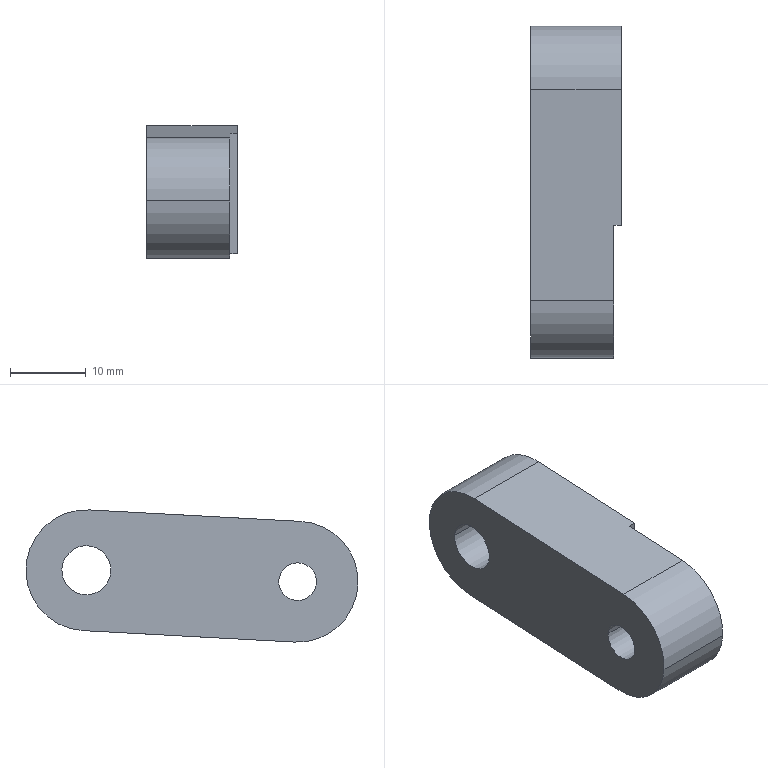Component | SolidWorks | NewDieSet-1_AdditionalStop-2 | 1 solid | 13 faces | box 12 x 43.96 x 17.51 mm | volume 6914 mm3 | cylinder 7 | plane 6 | commonest cylinder face diameters 16 x3 5 x2 6.5 x2
build123d program:
from build123d import *

# Parameters (mm, degrees)
BOSS_EXTRUDE1_DEPTH = 12
SKETCH2_R           = 3.25
CUT_EXTRUDE1_DEPTH  = 12
M6_TAPPED_HOLE1_D   = 5
SKETCH6_W           = 18
SKETCH6_H           = 1
CUT_EXTRUDE2_DEPTH  = 30.732


with BuildPart() as part:
    # Sketch1 → Boss-Extrude1 (new body)
    with BuildSketch(Plane(origin=(0, 0, 0), x_dir=(1, 0, 0), z_dir=(0, 1, 0))):
        with BuildLine():
            Line((-8, -14), (-8, 14))
            ThreePointArc((-8, 14), (0, 22), (8, 14))
            Line((8, 14), (8, -14))
            ThreePointArc((8, -14), (0, -22), (-8, -14))
        make_face()
    extrude(amount=BOSS_EXTRUDE1_DEPTH)

    # Sketch2 → Cut-Extrude1 (cut)
    with BuildSketch(Plane(origin=(0, 12, 0), x_dir=(1, 0, 0), z_dir=(0, 1, 0))):
        with Locations(Location((0, -14, 0), (0, 0, 270))):
            Circle(SKETCH2_R)
    extrude(amount=-CUT_EXTRUDE1_DEPTH, mode=Mode.SUBTRACT)

    # M6 Tapped Hole1 (through all)
    with Locations(Plane(origin=(0, 12, 0), x_dir=(1, 0, 0), z_dir=(0, 1, 0))):
        with Locations((0, 14)):
            Hole(M6_TAPPED_HOLE1_D / 2)

    # Sketch6 → Cut-Extrude2 (cut, through all)
    with BuildSketch(Plane.ZY.offset(8)):
        with Locations((-13, 0.5)):
            Rectangle(SKETCH6_W, SKETCH6_H)
    extrude(amount=-CUT_EXTRUDE2_DEPTH, mode=Mode.SUBTRACT)


solid = part.part

# Placed as in the assembly
solid = solid.moved(Location((-256.746, 103.448, 192.243), (-86.9, 0, 90)))
STEP:
#1=COLOUR_RGB('',0.7922,0.8196,0.9333);
#2=FILL_AREA_STYLE_COLOUR('',#1);
#3=FILL_AREA_STYLE('',(#2));
#4=SURFACE_STYLE_FILL_AREA(#3);
#5=SURFACE_SIDE_STYLE('',(#4));
#6=SURFACE_STYLE_USAGE(.BOTH.,#5);
#7=PRESENTATION_STYLE_ASSIGNMENT((#6));
#8=CARTESIAN_POINT('',(-10.147,3.621,7.544));
#9=VERTEX_POINT('',#8);
#10=CARTESIAN_POINT('',(-10.147,3.424,7.533));
#11=VERTEX_POINT('',#10);
#12=CARTESIAN_POINT('',(-10.147,3.522,7.539));
#13=DIRECTION('',(1.,0.,0.));
#14=DIRECTION('',(0.,0.9985,0.05408));
#15=AXIS2_PLACEMENT_3D('',#12,#13,#14);
#16=CIRCLE('',#15,0.09843);
#17=EDGE_CURVE('',#9,#11,#16,.T.);
#18=ORIENTED_EDGE('',*,*,#17,.T.);
#19=CARTESIAN_POINT('',(-10.581,3.424,7.533));
#20=VERTEX_POINT('',#19);
#21=CARTESIAN_POINT('',(-10.581,3.424,7.533));
#22=DIRECTION('',(-1.,0.,0.));
#23=VECTOR('',#22,39.37);
#24=LINE('',#21,#23);
#25=EDGE_CURVE('',#11,#20,#24,.T.);
#26=ORIENTED_EDGE('',*,*,#25,.T.);
#27=CARTESIAN_POINT('',(-10.581,3.621,7.544));
#28=VERTEX_POINT('',#27);
#29=CARTESIAN_POINT('',(-10.581,3.522,7.539));
#30=DIRECTION('',(-1.,0.,0.));
#31=DIRECTION('',(0.,0.9985,0.05408));
#32=AXIS2_PLACEMENT_3D('',#29,#30,#31);
#33=CIRCLE('',#32,0.09843);
#34=EDGE_CURVE('',#20,#28,#33,.T.);
#35=ORIENTED_EDGE('',*,*,#34,.T.);
#36=CARTESIAN_POINT('',(-10.581,3.621,7.544));
#37=DIRECTION('',(-1.,0.,0.));
#38=VECTOR('',#37,39.37);
#39=LINE('',#36,#38);
#40=EDGE_CURVE('',#9,#28,#39,.T.);
#41=ORIENTED_EDGE('',*,*,#40,.F.);
#42=EDGE_LOOP('',(#18,#26,#35,#41));
#43=FACE_OUTER_BOUND('',#42,.T.);
#44=CARTESIAN_POINT('',(-10.581,3.522,7.539));
#45=DIRECTION('',(-1.,0.,0.));
#46=DIRECTION('',(0.,0.9985,0.05408));
#47=AXIS2_PLACEMENT_3D('',#44,#45,#46);
#48=CYLINDRICAL_SURFACE('',#47,0.09843);
#49=ADVANCED_FACE('',(#43),#48,.F.);
#50=CARTESIAN_POINT('',(-10.108,4.495,7.592));
#51=VERTEX_POINT('',#50);
#52=CARTESIAN_POINT('',(-10.108,4.751,7.605));
#53=VERTEX_POINT('',#52);
#54=CARTESIAN_POINT('',(-10.108,4.623,7.598));
#55=DIRECTION('',(-1.,0.,0.));
#56=DIRECTION('',(0.,0.9985,0.05408));
#57=AXIS2_PLACEMENT_3D('',#54,#55,#56);
#58=CIRCLE('',#57,0.128);
#59=EDGE_CURVE('',#51,#53,#58,.T.);
#60=ORIENTED_EDGE('',*,*,#59,.F.);
#61=CARTESIAN_POINT('',(-10.581,4.495,7.592));
#62=VERTEX_POINT('',#61);
#63=CARTESIAN_POINT('',(-10.108,4.495,7.592));
#64=DIRECTION('',(-1.,0.,0.));
#65=VECTOR('',#64,39.37);
#66=LINE('',#63,#65);
#67=EDGE_CURVE('',#51,#62,#66,.T.);
#68=ORIENTED_EDGE('',*,*,#67,.T.);
#69=CARTESIAN_POINT('',(-10.581,4.751,7.605));
#70=VERTEX_POINT('',#69);
#71=CARTESIAN_POINT('',(-10.581,4.623,7.598));
#72=DIRECTION('',(-1.,0.,0.));
#73=DIRECTION('',(0.,0.9985,0.05408));
#74=AXIS2_PLACEMENT_3D('',#71,#72,#73);
#75=CIRCLE('',#74,0.128);
#76=EDGE_CURVE('',#62,#70,#75,.T.);
#77=ORIENTED_EDGE('',*,*,#76,.T.);
#78=CARTESIAN_POINT('',(-10.108,4.751,7.605));
#79=DIRECTION('',(-1.,0.,0.));
#80=VECTOR('',#79,39.37);
#81=LINE('',#78,#80);
#82=EDGE_CURVE('',#53,#70,#81,.T.);
#83=ORIENTED_EDGE('',*,*,#82,.F.);
#84=EDGE_LOOP('',(#60,#68,#77,#83));
#85=FACE_OUTER_BOUND('',#84,.T.);
#86=CARTESIAN_POINT('',(-10.108,4.623,7.598));
#87=DIRECTION('',(-1.,0.,0.));
#88=DIRECTION('',(0.,0.9985,0.05408));
#89=AXIS2_PLACEMENT_3D('',#86,#87,#88);
#90=CYLINDRICAL_SURFACE('',#89,0.128);
#91=ADVANCED_FACE('',(#85),#90,.F.);
#92=CARTESIAN_POINT('',(-10.581,3.208,7.522));
#93=VERTEX_POINT('',#92);
#94=CARTESIAN_POINT('',(-10.581,3.505,7.853));
#95=VERTEX_POINT('',#94);
#96=CARTESIAN_POINT('',(-10.581,3.522,7.539));
#97=DIRECTION('',(-1.,0.,0.));
#98=DIRECTION('',(0.,0.9985,0.05408));
#99=AXIS2_PLACEMENT_3D('',#96,#97,#98);
#100=CIRCLE('',#99,0.315);
#101=EDGE_CURVE('',#93,#95,#100,.T.);
#102=ORIENTED_EDGE('',*,*,#101,.F.);
#103=CARTESIAN_POINT('',(-10.147,3.208,7.522));
#104=VERTEX_POINT('',#103);
#105=CARTESIAN_POINT('',(-10.581,3.208,7.522));
#106=DIRECTION('',(1.,0.,0.));
#107=VECTOR('',#106,39.37);
#108=LINE('',#105,#107);
#109=EDGE_CURVE('',#93,#104,#108,.T.);
#110=ORIENTED_EDGE('',*,*,#109,.T.);
#111=CARTESIAN_POINT('',(-10.147,3.505,7.853));
#112=VERTEX_POINT('',#111);
#113=CARTESIAN_POINT('',(-10.147,3.522,7.539));
#114=DIRECTION('',(-1.,0.,0.));
#115=DIRECTION('',(0.,0.9985,0.05408));
#116=AXIS2_PLACEMENT_3D('',#113,#114,#115);
#117=CIRCLE('',#116,0.315);
#118=EDGE_CURVE('',#104,#112,#117,.T.);
#119=ORIENTED_EDGE('',*,*,#118,.T.);
#120=CARTESIAN_POINT('',(-10.581,3.505,7.853));
#121=DIRECTION('',(1.,0.,0.));
#122=VECTOR('',#121,39.37);
#123=LINE('',#120,#122);
#124=EDGE_CURVE('',#95,#112,#123,.T.);
#125=ORIENTED_EDGE('',*,*,#124,.F.);
#126=EDGE_LOOP('',(#102,#110,#119,#125));
#127=FACE_OUTER_BOUND('',#126,.T.);
#128=CARTESIAN_POINT('',(-10.581,3.522,7.539));
#129=DIRECTION('',(1.,0.,0.));
#130=DIRECTION('',(0.,-0.9985,-0.05408));
#131=AXIS2_PLACEMENT_3D('',#128,#129,#130);
#132=CYLINDRICAL_SURFACE('',#131,0.315);
#133=ADVANCED_FACE('',(#127),#132,.T.);
#134=CARTESIAN_POINT('',(-10.108,4.606,7.913));
#135=VERTEX_POINT('',#134);
#136=CARTESIAN_POINT('',(-10.108,4.64,7.284));
#137=VERTEX_POINT('',#136);
#138=CARTESIAN_POINT('',(-10.108,4.623,7.598));
#139=DIRECTION('',(-1.,0.,0.));
#140=DIRECTION('',(0.,0.9985,0.05408));
#141=AXIS2_PLACEMENT_3D('',#138,#139,#140);
#142=CIRCLE('',#141,0.315);
#143=EDGE_CURVE('',#135,#137,#142,.T.);
#144=ORIENTED_EDGE('',*,*,#143,.T.);
#145=CARTESIAN_POINT('',(-10.581,4.64,7.284));
#146=VERTEX_POINT('',#145);
#147=CARTESIAN_POINT('',(-10.581,4.64,7.284));
#148=DIRECTION('',(1.,0.,0.));
#149=VECTOR('',#148,39.37);
#150=LINE('',#147,#149);
#151=EDGE_CURVE('',#146,#137,#150,.T.);
#152=ORIENTED_EDGE('',*,*,#151,.F.);
#153=CARTESIAN_POINT('',(-10.581,4.606,7.913));
#154=VERTEX_POINT('',#153);
#155=CARTESIAN_POINT('',(-10.581,4.623,7.598));
#156=DIRECTION('',(-1.,0.,0.));
#157=DIRECTION('',(0.,0.9985,0.05408));
#158=AXIS2_PLACEMENT_3D('',#155,#156,#157);
#159=CIRCLE('',#158,0.315);
#160=EDGE_CURVE('',#154,#146,#159,.T.);
#161=ORIENTED_EDGE('',*,*,#160,.F.);
#162=CARTESIAN_POINT('',(-10.581,4.606,7.913));
#163=DIRECTION('',(1.,0.,0.));
#164=VECTOR('',#163,39.37);
#165=LINE('',#162,#164);
#166=EDGE_CURVE('',#154,#135,#165,.T.);
#167=ORIENTED_EDGE('',*,*,#166,.T.);
#168=EDGE_LOOP('',(#144,#152,#161,#167));
#169=FACE_OUTER_BOUND('',#168,.T.);
#170=CARTESIAN_POINT('',(-10.581,4.623,7.598));
#171=DIRECTION('',(1.,0.,0.));
#172=DIRECTION('',(0.,-0.9985,-0.05408));
#173=AXIS2_PLACEMENT_3D('',#170,#171,#172);
#174=CYLINDRICAL_SURFACE('',#173,0.315);
#175=ADVANCED_FACE('',(#169),#174,.T.);
#176=CARTESIAN_POINT('',(-10.108,3.933,7.246));
#177=VERTEX_POINT('',#176);
#178=CARTESIAN_POINT('',(-10.147,3.933,7.246));
#179=VERTEX_POINT('',#178);
#180=CARTESIAN_POINT('',(-10.108,3.933,7.246));
#181=DIRECTION('',(-1.,0.,0.));
#182=VECTOR('',#181,39.37);
#183=LINE('',#180,#182);
#184=EDGE_CURVE('',#177,#179,#183,.T.);
#185=ORIENTED_EDGE('',*,*,#184,.T.);
#186=CARTESIAN_POINT('',(-10.147,3.539,7.224));
#187=VERTEX_POINT('',#186);
#188=CARTESIAN_POINT('',(-10.147,3.225,7.207));
#189=DIRECTION('',(0.,-0.9985,-0.05408));
#190=VECTOR('',#189,39.37);
#191=LINE('',#188,#190);
#192=EDGE_CURVE('',#179,#187,#191,.T.);
#193=ORIENTED_EDGE('',*,*,#192,.T.);
#194=CARTESIAN_POINT('',(-10.581,3.539,7.224));
#195=VERTEX_POINT('',#194);
#196=CARTESIAN_POINT('',(-10.581,3.539,7.224));
#197=DIRECTION('',(1.,0.,0.));
#198=VECTOR('',#197,39.37);
#199=LINE('',#196,#198);
#200=EDGE_CURVE('',#195,#187,#199,.T.);
#201=ORIENTED_EDGE('',*,*,#200,.F.);
#202=CARTESIAN_POINT('',(-10.581,4.64,7.284));
#203=DIRECTION('',(0.,-0.9985,-0.05408));
#204=VECTOR('',#203,39.37);
#205=LINE('',#202,#204);
#206=EDGE_CURVE('',#146,#195,#205,.T.);
#207=ORIENTED_EDGE('',*,*,#206,.F.);
#208=ORIENTED_EDGE('',*,*,#151,.T.);
#209=CARTESIAN_POINT('',(-10.108,4.64,7.284));
#210=DIRECTION('',(0.,-0.9985,-0.05408));
#211=VECTOR('',#210,39.37);
#212=LINE('',#209,#211);
#213=EDGE_CURVE('',#137,#177,#212,.T.);
#214=ORIENTED_EDGE('',*,*,#213,.T.);
#215=EDGE_LOOP('',(#185,#193,#201,#207,#208,#214));
#216=FACE_OUTER_BOUND('',#215,.T.);
#217=CARTESIAN_POINT('',(-10.581,4.64,7.284));
#218=DIRECTION('',(0.,-0.05408,0.9985));
#219=DIRECTION('',(0.,0.9985,0.05408));
#220=AXIS2_PLACEMENT_3D('',#217,#218,#219);
#221=PLANE('',#220);
#222=ADVANCED_FACE('',(#216),#221,.F.);
#223=ORIENTED_EDGE('',*,*,#109,.F.);
#224=CARTESIAN_POINT('',(-10.581,3.522,7.539));
#225=DIRECTION('',(-1.,0.,0.));
#226=DIRECTION('',(0.,0.9985,0.05408));
#227=AXIS2_PLACEMENT_3D('',#224,#225,#226);
#228=CIRCLE('',#227,0.315);
#229=EDGE_CURVE('',#195,#93,#228,.T.);
#230=ORIENTED_EDGE('',*,*,#229,.F.);
#231=ORIENTED_EDGE('',*,*,#200,.T.);
#232=CARTESIAN_POINT('',(-10.147,3.522,7.539));
#233=DIRECTION('',(-1.,0.,0.));
#234=DIRECTION('',(0.,0.9985,0.05408));
#235=AXIS2_PLACEMENT_3D('',#232,#233,#234);
#236=CIRCLE('',#235,0.315);
#237=EDGE_CURVE('',#187,#104,#236,.T.);
#238=ORIENTED_EDGE('',*,*,#237,.T.);
#239=EDGE_LOOP('',(#223,#230,#231,#238));
#240=FACE_OUTER_BOUND('',#239,.T.);
#241=CARTESIAN_POINT('',(-10.581,3.522,7.539));
#242=DIRECTION('',(1.,0.,0.));
#243=DIRECTION('',(0.,-0.9985,-0.05408));
#244=AXIS2_PLACEMENT_3D('',#241,#242,#243);
#245=CYLINDRICAL_SURFACE('',#244,0.315);
#246=ADVANCED_FACE('',(#240),#245,.T.);
#247=ORIENTED_EDGE('',*,*,#124,.T.);
#248=CARTESIAN_POINT('',(-10.147,3.898,7.875));
#249=VERTEX_POINT('',#248);
#250=CARTESIAN_POINT('',(-10.147,3.191,7.836));
#251=DIRECTION('',(0.,-0.9985,-0.05408));
#252=VECTOR('',#251,39.37);
#253=LINE('',#250,#252);
#254=EDGE_CURVE('',#249,#112,#253,.T.);
#255=ORIENTED_EDGE('',*,*,#254,.F.);
#256=CARTESIAN_POINT('',(-10.108,3.898,7.875));
#257=VERTEX_POINT('',#256);
#258=CARTESIAN_POINT('',(-10.108,3.898,7.875));
#259=DIRECTION('',(-1.,0.,0.));
#260=VECTOR('',#259,39.37);
#261=LINE('',#258,#260);
#262=EDGE_CURVE('',#257,#249,#261,.T.);
#263=ORIENTED_EDGE('',*,*,#262,.F.);
#264=CARTESIAN_POINT('',(-10.108,4.606,7.913));
#265=DIRECTION('',(0.,0.9985,0.05408));
#266=VECTOR('',#265,39.37);
#267=LINE('',#264,#266);
#268=EDGE_CURVE('',#257,#135,#267,.T.);
#269=ORIENTED_EDGE('',*,*,#268,.T.);
#270=ORIENTED_EDGE('',*,*,#166,.F.);
#271=CARTESIAN_POINT('',(-10.581,4.606,7.913));
#272=DIRECTION('',(0.,0.9985,0.05408));
#273=VECTOR('',#272,39.37);
#274=LINE('',#271,#273);
#275=EDGE_CURVE('',#95,#154,#274,.T.);
#276=ORIENTED_EDGE('',*,*,#275,.F.);
#277=EDGE_LOOP('',(#247,#255,#263,#269,#270,#276));
#278=FACE_OUTER_BOUND('',#277,.T.);
#279=CARTESIAN_POINT('',(-10.581,4.606,7.913));
#280=DIRECTION('',(0.,0.05408,-0.9985));
#281=DIRECTION('',(0.,-0.9985,-0.05408));
#282=AXIS2_PLACEMENT_3D('',#279,#280,#281);
#283=PLANE('',#282);
#284=ADVANCED_FACE('',(#278),#283,.F.);
#285=CARTESIAN_POINT('',(-10.581,3.522,7.539));
#286=DIRECTION('',(-1.,0.,0.));
#287=DIRECTION('',(0.,0.9985,0.05408));
#288=AXIS2_PLACEMENT_3D('',#285,#286,#287);
#289=CIRCLE('',#288,0.09843);
#290=EDGE_CURVE('',#28,#20,#289,.T.);
#291=ORIENTED_EDGE('',*,*,#290,.F.);
#292=ORIENTED_EDGE('',*,*,#34,.F.);
#293=EDGE_LOOP('',(#291,#292));
#294=FACE_BOUND('',#293,.T.);
#295=CARTESIAN_POINT('',(-10.581,4.623,7.598));
#296=DIRECTION('',(-1.,0.,0.));
#297=DIRECTION('',(0.,0.9985,0.05408));
#298=AXIS2_PLACEMENT_3D('',#295,#296,#297);
#299=CIRCLE('',#298,0.128);
#300=EDGE_CURVE('',#70,#62,#299,.T.);
#301=ORIENTED_EDGE('',*,*,#300,.F.);
#302=ORIENTED_EDGE('',*,*,#76,.F.);
#303=EDGE_LOOP('',(#301,#302));
#304=FACE_BOUND('',#303,.T.);
#305=ORIENTED_EDGE('',*,*,#160,.T.);
#306=ORIENTED_EDGE('',*,*,#206,.T.);
#307=ORIENTED_EDGE('',*,*,#229,.T.);
#308=ORIENTED_EDGE('',*,*,#101,.T.);
#309=ORIENTED_EDGE('',*,*,#275,.T.);
#310=EDGE_LOOP('',(#305,#306,#307,#308,#309));
#311=FACE_OUTER_BOUND('',#310,.T.);
#312=CARTESIAN_POINT('',(-10.581,4.623,7.598));
#313=DIRECTION('',(-1.,0.,0.));
#314=DIRECTION('',(0.,0.9985,0.05408));
#315=AXIS2_PLACEMENT_3D('',#312,#313,#314);
#316=PLANE('',#315);
#317=ADVANCED_FACE('',(#294,#304,#311),#316,.T.);
#318=CARTESIAN_POINT('',(-10.108,4.623,7.598));
#319=DIRECTION('',(-1.,0.,0.));
#320=DIRECTION('',(0.,0.9985,0.05408));
#321=AXIS2_PLACEMENT_3D('',#318,#319,#320);
#322=CIRCLE('',#321,0.128);
#323=EDGE_CURVE('',#53,#51,#322,.T.);
#324=ORIENTED_EDGE('',*,*,#323,.T.);
#325=ORIENTED_EDGE('',*,*,#59,.T.);
#326=EDGE_LOOP('',(#324,#325));
#327=FACE_BOUND('',#326,.T.);
#328=ORIENTED_EDGE('',*,*,#268,.F.);
#329=CARTESIAN_POINT('',(-10.108,3.933,7.246));
#330=DIRECTION('',(0.,-0.05408,0.9985));
#331=VECTOR('',#330,39.37);
#332=LINE('',#329,#331);
#333=EDGE_CURVE('',#177,#257,#332,.T.);
#334=ORIENTED_EDGE('',*,*,#333,.F.);
#335=ORIENTED_EDGE('',*,*,#213,.F.);
#336=ORIENTED_EDGE('',*,*,#143,.F.);
#337=EDGE_LOOP('',(#328,#334,#335,#336));
#338=FACE_OUTER_BOUND('',#337,.T.);
#339=CARTESIAN_POINT('',(-10.108,4.623,7.598));
#340=DIRECTION('',(-1.,0.,0.));
#341=DIRECTION('',(0.,0.9985,0.05408));
#342=AXIS2_PLACEMENT_3D('',#339,#340,#341);
#343=PLANE('',#342);
#344=ADVANCED_FACE('',(#327,#338),#343,.F.);
#345=ORIENTED_EDGE('',*,*,#67,.F.);
#346=ORIENTED_EDGE('',*,*,#323,.F.);
#347=ORIENTED_EDGE('',*,*,#82,.T.);
#348=ORIENTED_EDGE('',*,*,#300,.T.);
#349=EDGE_LOOP('',(#345,#346,#347,#348));
#350=FACE_OUTER_BOUND('',#349,.T.);
#351=CARTESIAN_POINT('',(-10.108,4.623,7.598));
#352=DIRECTION('',(-1.,0.,0.));
#353=DIRECTION('',(0.,0.9985,0.05408));
#354=AXIS2_PLACEMENT_3D('',#351,#352,#353);
#355=CYLINDRICAL_SURFACE('',#354,0.128);
#356=ADVANCED_FACE('',(#350),#355,.F.);
#357=ORIENTED_EDGE('',*,*,#25,.F.);
#358=CARTESIAN_POINT('',(-10.147,3.522,7.539));
#359=DIRECTION('',(1.,0.,0.));
#360=DIRECTION('',(0.,0.9985,0.05408));
#361=AXIS2_PLACEMENT_3D('',#358,#359,#360);
#362=CIRCLE('',#361,0.09843);
#363=EDGE_CURVE('',#11,#9,#362,.T.);
#364=ORIENTED_EDGE('',*,*,#363,.T.);
#365=ORIENTED_EDGE('',*,*,#40,.T.);
#366=ORIENTED_EDGE('',*,*,#290,.T.);
#367=EDGE_LOOP('',(#357,#364,#365,#366));
#368=FACE_OUTER_BOUND('',#367,.T.);
#369=CARTESIAN_POINT('',(-10.581,3.522,7.539));
#370=DIRECTION('',(-1.,0.,0.));
#371=DIRECTION('',(0.,0.9985,0.05408));
#372=AXIS2_PLACEMENT_3D('',#369,#370,#371);
#373=CYLINDRICAL_SURFACE('',#372,0.09843);
#374=ADVANCED_FACE('',(#368),#373,.F.);
#375=ORIENTED_EDGE('',*,*,#17,.F.);
#376=ORIENTED_EDGE('',*,*,#363,.F.);
#377=EDGE_LOOP('',(#375,#376));
#378=FACE_BOUND('',#377,.T.);
#379=ORIENTED_EDGE('',*,*,#192,.F.);
#380=CARTESIAN_POINT('',(-10.147,3.933,7.246));
#381=DIRECTION('',(0.,-0.05408,0.9985));
#382=VECTOR('',#381,39.37);
#383=LINE('',#380,#382);
#384=EDGE_CURVE('',#179,#249,#383,.T.);
#385=ORIENTED_EDGE('',*,*,#384,.T.);
#386=ORIENTED_EDGE('',*,*,#254,.T.);
#387=ORIENTED_EDGE('',*,*,#118,.F.);
#388=ORIENTED_EDGE('',*,*,#237,.F.);
#389=EDGE_LOOP('',(#379,#385,#386,#387,#388));
#390=FACE_OUTER_BOUND('',#389,.T.);
#391=CARTESIAN_POINT('',(-10.147,3.225,7.207));
#392=DIRECTION('',(-1.,0.,0.));
#393=DIRECTION('',(0.,0.9985,0.05408));
#394=AXIS2_PLACEMENT_3D('',#391,#392,#393);
#395=PLANE('',#394);
#396=ADVANCED_FACE('',(#378,#390),#395,.F.);
#397=ORIENTED_EDGE('',*,*,#262,.T.);
#398=ORIENTED_EDGE('',*,*,#384,.F.);
#399=ORIENTED_EDGE('',*,*,#184,.F.);
#400=ORIENTED_EDGE('',*,*,#333,.T.);
#401=EDGE_LOOP('',(#397,#398,#399,#400));
#402=FACE_OUTER_BOUND('',#401,.T.);
#403=CARTESIAN_POINT('',(-10.108,3.933,7.246));
#404=DIRECTION('',(0.,0.9985,0.05408));
#405=DIRECTION('',(0.,0.05408,-0.9985));
#406=AXIS2_PLACEMENT_3D('',#403,#404,#405);
#407=PLANE('',#406);
#408=ADVANCED_FACE('',(#402),#407,.F.);
#409=CLOSED_SHELL('',(#49,#91,#133,#175,#222,#246,#284,#317,#344,#356,#374,#396,#408));
#410=MANIFOLD_SOLID_BREP('',#409);
#411=STYLED_ITEM('',(#7),#410);
#412=(LENGTH_UNIT()NAMED_UNIT(*)SI_UNIT($,.METRE.));
#413=LENGTH_MEASURE_WITH_UNIT(LENGTH_MEASURE(0.0254),#412);
#414=DIMENSIONAL_EXPONENTS(1.,0.,0.,0.,0.,0.,0.);
#415=(CONVERSION_BASED_UNIT('',#413)LENGTH_UNIT()NAMED_UNIT(#414));
#416=UNCERTAINTY_MEASURE_WITH_UNIT(LENGTH_MEASURE(0.00001),#415,'','');
#417=(NAMED_UNIT(*)PLANE_ANGLE_UNIT()SI_UNIT($,.RADIAN.));
#418=(NAMED_UNIT(*)SI_UNIT($,.STERADIAN.)SOLID_ANGLE_UNIT());
#419=(GEOMETRIC_REPRESENTATION_CONTEXT(3)GLOBAL_UNCERTAINTY_ASSIGNED_CONTEXT((#416))GLOBAL_UNIT_ASSIGNED_CONTEXT((#415,#417,#418))REPRESENTATION_CONTEXT('',''));
#420=MECHANICAL_DESIGN_GEOMETRIC_PRESENTATION_REPRESENTATION('',(#411),#419);
#421=CARTESIAN_POINT('',(0.,0.,0.));
#422=DIRECTION('',(0.,0.,1.));
#423=DIRECTION('',(1.,0.,0.));
#424=AXIS2_PLACEMENT_3D('',#421,#422,#423);
#425=(LENGTH_UNIT()NAMED_UNIT(*)SI_UNIT($,.METRE.));
#426=LENGTH_MEASURE_WITH_UNIT(LENGTH_MEASURE(0.0254),#425);
#427=DIMENSIONAL_EXPONENTS(1.,0.,0.,0.,0.,0.,0.);
#428=(CONVERSION_BASED_UNIT('',#426)LENGTH_UNIT()NAMED_UNIT(#427));
#429=UNCERTAINTY_MEASURE_WITH_UNIT(LENGTH_MEASURE(0.00001),#428,'','');
#430=(NAMED_UNIT(*)PLANE_ANGLE_UNIT()SI_UNIT($,.RADIAN.));
#431=(NAMED_UNIT(*)SI_UNIT($,.STERADIAN.)SOLID_ANGLE_UNIT());
#432=(GEOMETRIC_REPRESENTATION_CONTEXT(3)GLOBAL_UNCERTAINTY_ASSIGNED_CONTEXT((#429))GLOBAL_UNIT_ASSIGNED_CONTEXT((#428,#430,#431))REPRESENTATION_CONTEXT('',''));
#433=ADVANCED_BREP_SHAPE_REPRESENTATION('',(#410,#424),#432);
#434=PRESENTATION_LAYER_ASSIGNMENT('','',(#411));